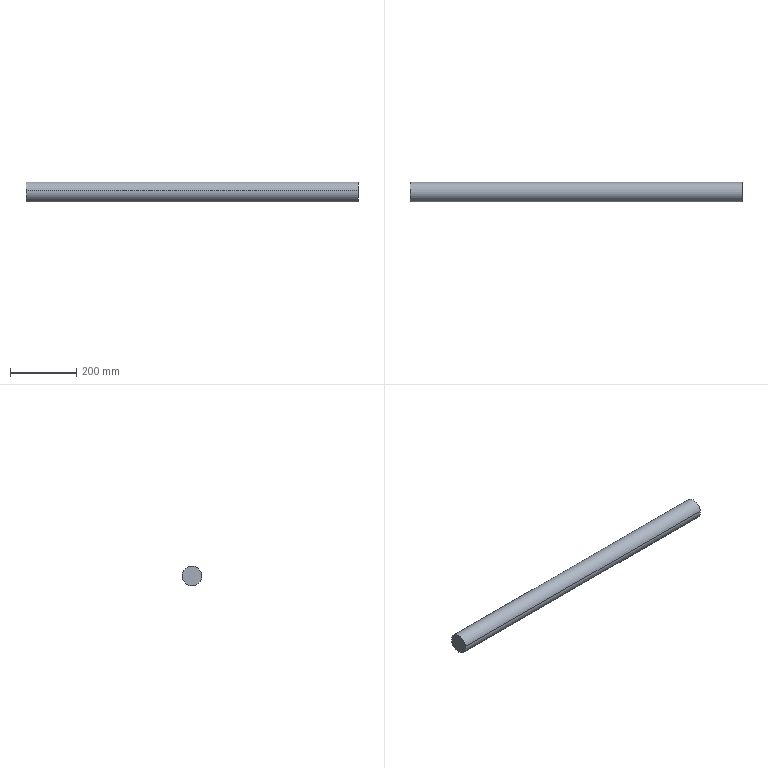Component | SolidWorks | Assembly2-1_Crossbeam-1 | 1 solid | 4 faces | box 1000 x 60 x 60 mm | volume 2827433 mm3 | cylinder 2 | plane 2 | commonest cylinder face diameters 60 x2
build123d program:
from build123d import *

# Parameters (mm, degrees)
SKETCH1_R           = 30
BOSS_EXTRUDE1_DEPTH = 1000


with BuildPart() as part:
    # Sketch1 → Boss-Extrude1 (new body)
    with BuildSketch(Plane.XY):
        Circle(SKETCH1_R)
    extrude(amount=BOSS_EXTRUDE1_DEPTH)


solid = part.part

# Placed as in the assembly
solid = solid.moved(Location((-653.02, 275.819, 0), (0, 90, 0)))
STEP:
#1=COLOUR_RGB('',0.7922,0.8196,0.9333);
#2=FILL_AREA_STYLE_COLOUR('',#1);
#3=FILL_AREA_STYLE('',(#2));
#4=SURFACE_STYLE_FILL_AREA(#3);
#5=SURFACE_SIDE_STYLE('',(#4));
#6=SURFACE_STYLE_USAGE(.BOTH.,#5);
#7=PRESENTATION_STYLE_ASSIGNMENT((#6));
#8=CARTESIAN_POINT('',(13.661,12.025,-0.1891));
#9=VERTEX_POINT('',#8);
#10=CARTESIAN_POINT('',(13.661,9.693,0.1891));
#11=VERTEX_POINT('',#10);
#12=CARTESIAN_POINT('',(13.661,10.859,0.));
#13=DIRECTION('',(1.,0.,0.));
#14=DIRECTION('',(0.,0.9871,-0.1601));
#15=AXIS2_PLACEMENT_3D('',#12,#13,#14);
#16=CIRCLE('',#15,1.181);
#17=EDGE_CURVE('',#9,#11,#16,.T.);
#18=ORIENTED_EDGE('',*,*,#17,.F.);
#19=CARTESIAN_POINT('',(-25.709,12.025,-0.1891));
#20=VERTEX_POINT('',#19);
#21=CARTESIAN_POINT('',(13.661,12.025,-0.1891));
#22=DIRECTION('',(-1.,0.,0.));
#23=VECTOR('',#22,39.37);
#24=LINE('',#21,#23);
#25=EDGE_CURVE('',#9,#20,#24,.T.);
#26=ORIENTED_EDGE('',*,*,#25,.T.);
#27=CARTESIAN_POINT('',(-25.709,9.693,0.1891));
#28=VERTEX_POINT('',#27);
#29=CARTESIAN_POINT('',(-25.709,10.859,0.));
#30=DIRECTION('',(1.,0.,0.));
#31=DIRECTION('',(0.,0.9871,-0.1601));
#32=AXIS2_PLACEMENT_3D('',#29,#30,#31);
#33=CIRCLE('',#32,1.181);
#34=EDGE_CURVE('',#20,#28,#33,.T.);
#35=ORIENTED_EDGE('',*,*,#34,.T.);
#36=CARTESIAN_POINT('',(13.661,9.693,0.1891));
#37=DIRECTION('',(-1.,0.,0.));
#38=VECTOR('',#37,39.37);
#39=LINE('',#36,#38);
#40=EDGE_CURVE('',#11,#28,#39,.T.);
#41=ORIENTED_EDGE('',*,*,#40,.F.);
#42=EDGE_LOOP('',(#18,#26,#35,#41));
#43=FACE_OUTER_BOUND('',#42,.T.);
#44=CARTESIAN_POINT('',(13.661,10.859,0.));
#45=DIRECTION('',(-1.,0.,0.));
#46=DIRECTION('',(0.,-0.9871,0.1601));
#47=AXIS2_PLACEMENT_3D('',#44,#45,#46);
#48=CYLINDRICAL_SURFACE('',#47,1.181);
#49=ADVANCED_FACE('',(#43),#48,.T.);
#50=ORIENTED_EDGE('',*,*,#25,.F.);
#51=CARTESIAN_POINT('',(13.661,10.859,0.));
#52=DIRECTION('',(1.,0.,0.));
#53=DIRECTION('',(0.,0.9871,-0.1601));
#54=AXIS2_PLACEMENT_3D('',#51,#52,#53);
#55=CIRCLE('',#54,1.181);
#56=EDGE_CURVE('',#11,#9,#55,.T.);
#57=ORIENTED_EDGE('',*,*,#56,.F.);
#58=ORIENTED_EDGE('',*,*,#40,.T.);
#59=CARTESIAN_POINT('',(-25.709,10.859,0.));
#60=DIRECTION('',(1.,0.,0.));
#61=DIRECTION('',(0.,0.9871,-0.1601));
#62=AXIS2_PLACEMENT_3D('',#59,#60,#61);
#63=CIRCLE('',#62,1.181);
#64=EDGE_CURVE('',#28,#20,#63,.T.);
#65=ORIENTED_EDGE('',*,*,#64,.T.);
#66=EDGE_LOOP('',(#50,#57,#58,#65));
#67=FACE_OUTER_BOUND('',#66,.T.);
#68=CARTESIAN_POINT('',(13.661,10.859,0.));
#69=DIRECTION('',(-1.,0.,0.));
#70=DIRECTION('',(0.,-0.9871,0.1601));
#71=AXIS2_PLACEMENT_3D('',#68,#69,#70);
#72=CYLINDRICAL_SURFACE('',#71,1.181);
#73=ADVANCED_FACE('',(#67),#72,.T.);
#74=ORIENTED_EDGE('',*,*,#56,.T.);
#75=ORIENTED_EDGE('',*,*,#17,.T.);
#76=EDGE_LOOP('',(#74,#75));
#77=FACE_OUTER_BOUND('',#76,.T.);
#78=CARTESIAN_POINT('',(13.661,10.859,0.));
#79=DIRECTION('',(1.,0.,0.));
#80=DIRECTION('',(0.,0.9871,-0.1601));
#81=AXIS2_PLACEMENT_3D('',#78,#79,#80);
#82=PLANE('',#81);
#83=ADVANCED_FACE('',(#77),#82,.T.);
#84=ORIENTED_EDGE('',*,*,#64,.F.);
#85=ORIENTED_EDGE('',*,*,#34,.F.);
#86=EDGE_LOOP('',(#84,#85));
#87=FACE_OUTER_BOUND('',#86,.T.);
#88=CARTESIAN_POINT('',(-25.709,10.859,0.));
#89=DIRECTION('',(1.,0.,0.));
#90=DIRECTION('',(0.,0.9871,-0.1601));
#91=AXIS2_PLACEMENT_3D('',#88,#89,#90);
#92=PLANE('',#91);
#93=ADVANCED_FACE('',(#87),#92,.F.);
#94=CLOSED_SHELL('',(#49,#73,#83,#93));
#95=MANIFOLD_SOLID_BREP('',#94);
#96=STYLED_ITEM('',(#7),#95);
#97=(LENGTH_UNIT()NAMED_UNIT(*)SI_UNIT($,.METRE.));
#98=LENGTH_MEASURE_WITH_UNIT(LENGTH_MEASURE(0.0254),#97);
#99=DIMENSIONAL_EXPONENTS(1.,0.,0.,0.,0.,0.,0.);
#100=(CONVERSION_BASED_UNIT('',#98)LENGTH_UNIT()NAMED_UNIT(#99));
#101=UNCERTAINTY_MEASURE_WITH_UNIT(LENGTH_MEASURE(0.00001),#100,'','');
#102=(NAMED_UNIT(*)PLANE_ANGLE_UNIT()SI_UNIT($,.RADIAN.));
#103=(NAMED_UNIT(*)SI_UNIT($,.STERADIAN.)SOLID_ANGLE_UNIT());
#104=(GEOMETRIC_REPRESENTATION_CONTEXT(3)GLOBAL_UNCERTAINTY_ASSIGNED_CONTEXT((#101))GLOBAL_UNIT_ASSIGNED_CONTEXT((#100,#102,#103))REPRESENTATION_CONTEXT('',''));
#105=MECHANICAL_DESIGN_GEOMETRIC_PRESENTATION_REPRESENTATION('',(#96),#104);
#106=PRESENTATION_LAYER_ASSIGNMENT('','',(#96));
#107=CARTESIAN_POINT('',(0.,0.,0.));
#108=DIRECTION('',(0.,0.,1.));
#109=DIRECTION('',(1.,0.,0.));
#110=AXIS2_PLACEMENT_3D('',#107,#108,#109);
#111=(LENGTH_UNIT()NAMED_UNIT(*)SI_UNIT($,.METRE.));
#112=LENGTH_MEASURE_WITH_UNIT(LENGTH_MEASURE(0.0254),#111);
#113=DIMENSIONAL_EXPONENTS(1.,0.,0.,0.,0.,0.,0.);
#114=(CONVERSION_BASED_UNIT('',#112)LENGTH_UNIT()NAMED_UNIT(#113));
#115=UNCERTAINTY_MEASURE_WITH_UNIT(LENGTH_MEASURE(0.00001),#114,'','');
#116=(NAMED_UNIT(*)PLANE_ANGLE_UNIT()SI_UNIT($,.RADIAN.));
#117=(NAMED_UNIT(*)SI_UNIT($,.STERADIAN.)SOLID_ANGLE_UNIT());
#118=(GEOMETRIC_REPRESENTATION_CONTEXT(3)GLOBAL_UNCERTAINTY_ASSIGNED_CONTEXT((#115))GLOBAL_UNIT_ASSIGNED_CONTEXT((#114,#116,#117))REPRESENTATION_CONTEXT('',''));
#119=ADVANCED_BREP_SHAPE_REPRESENTATION('',(#95,#110),#118);